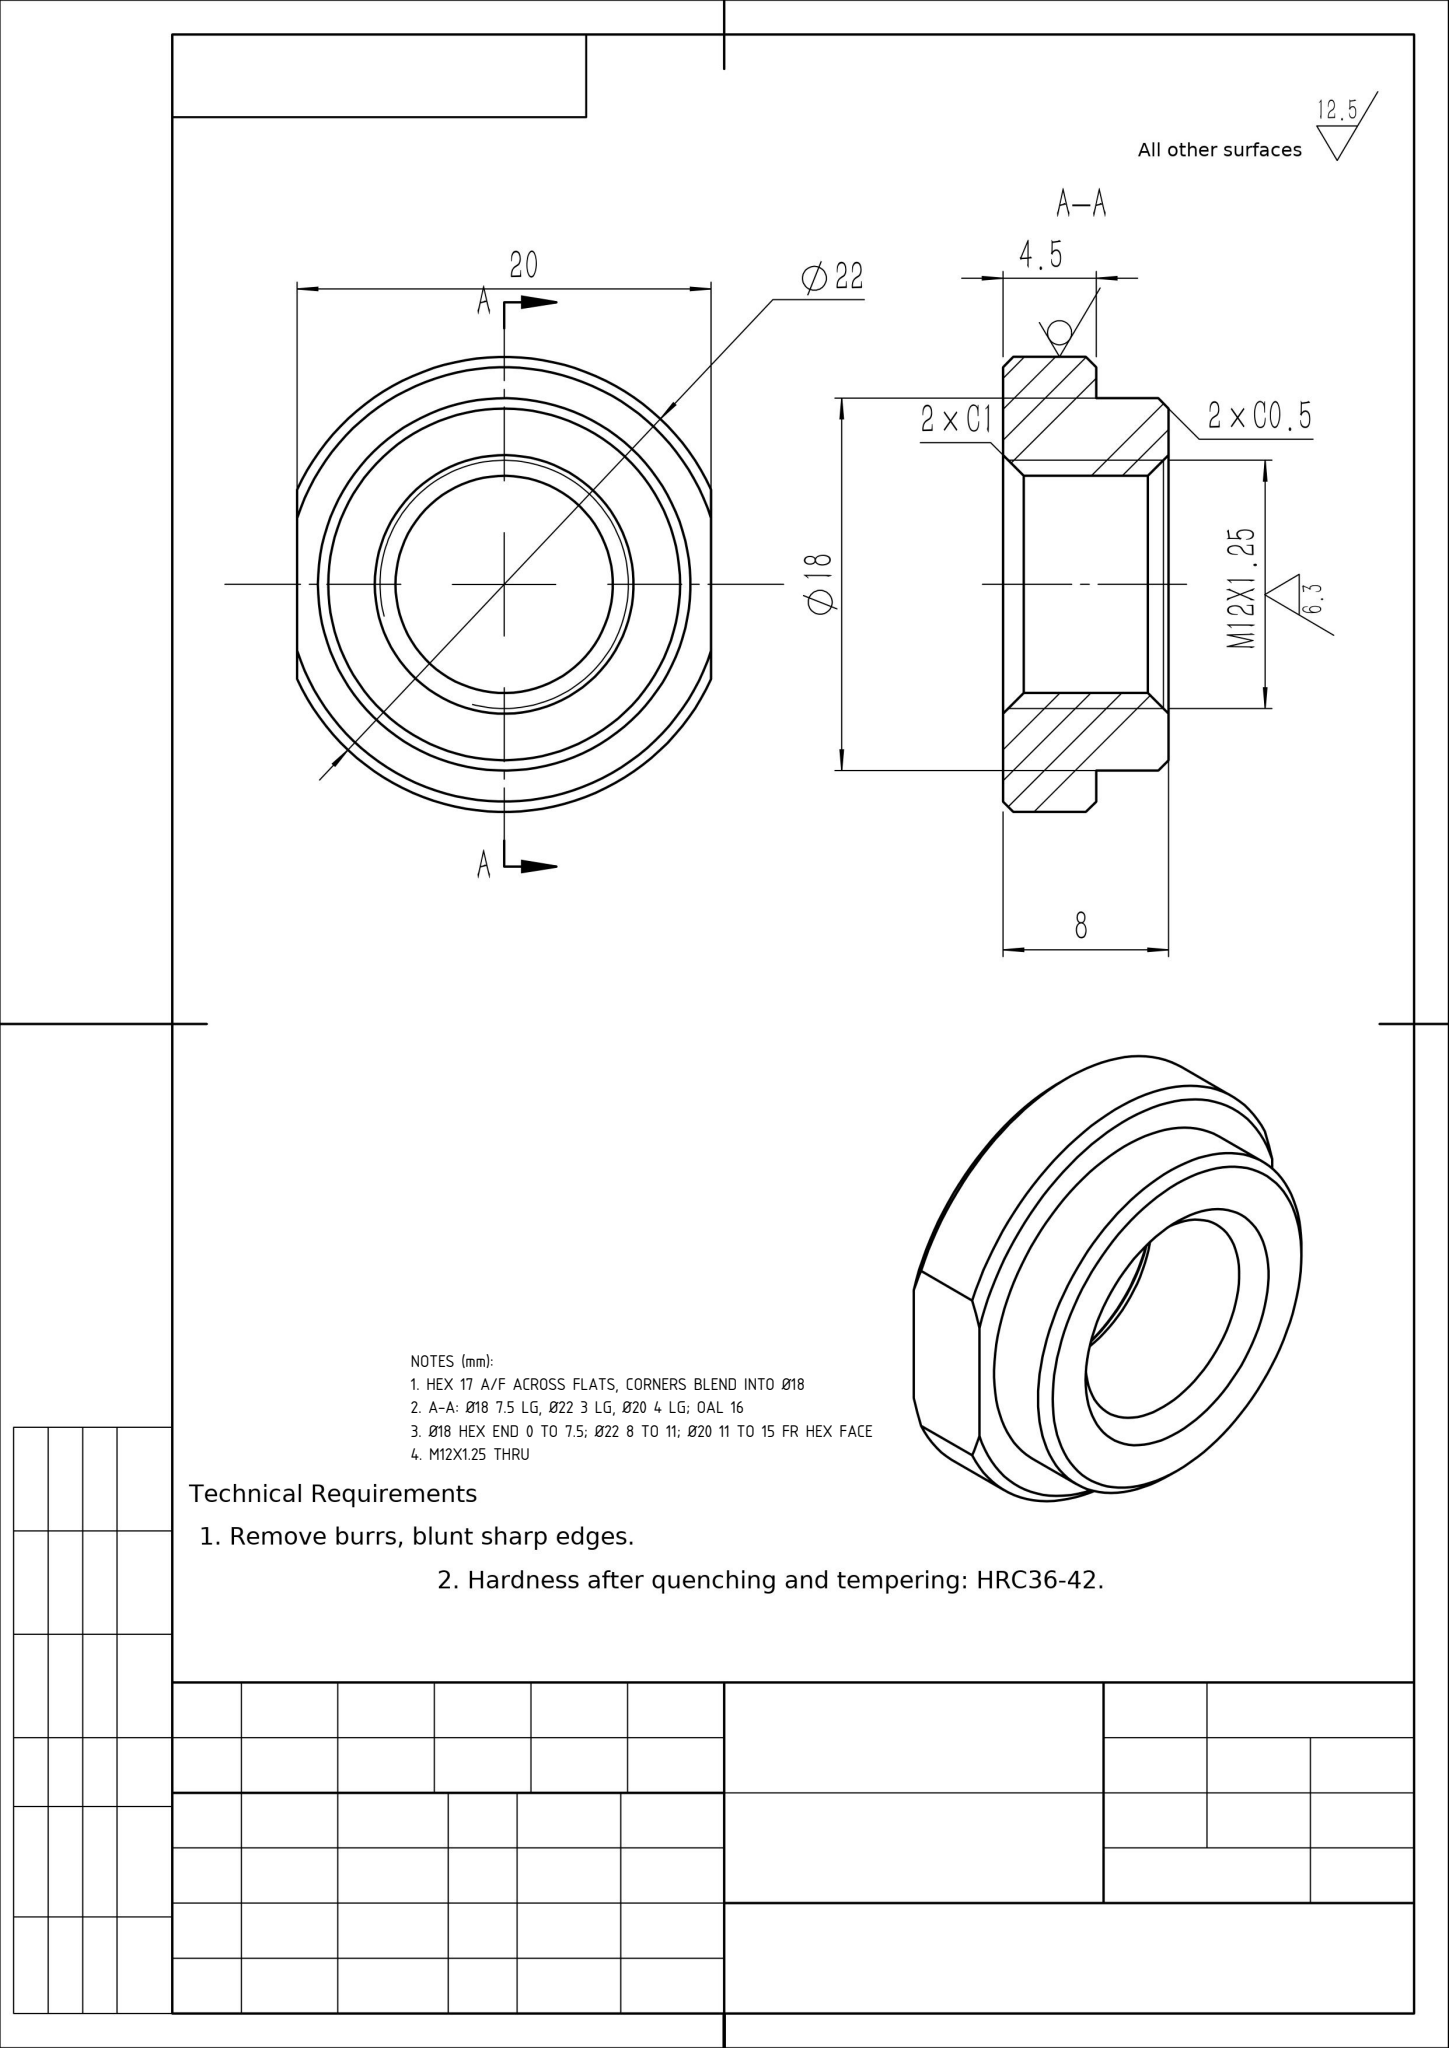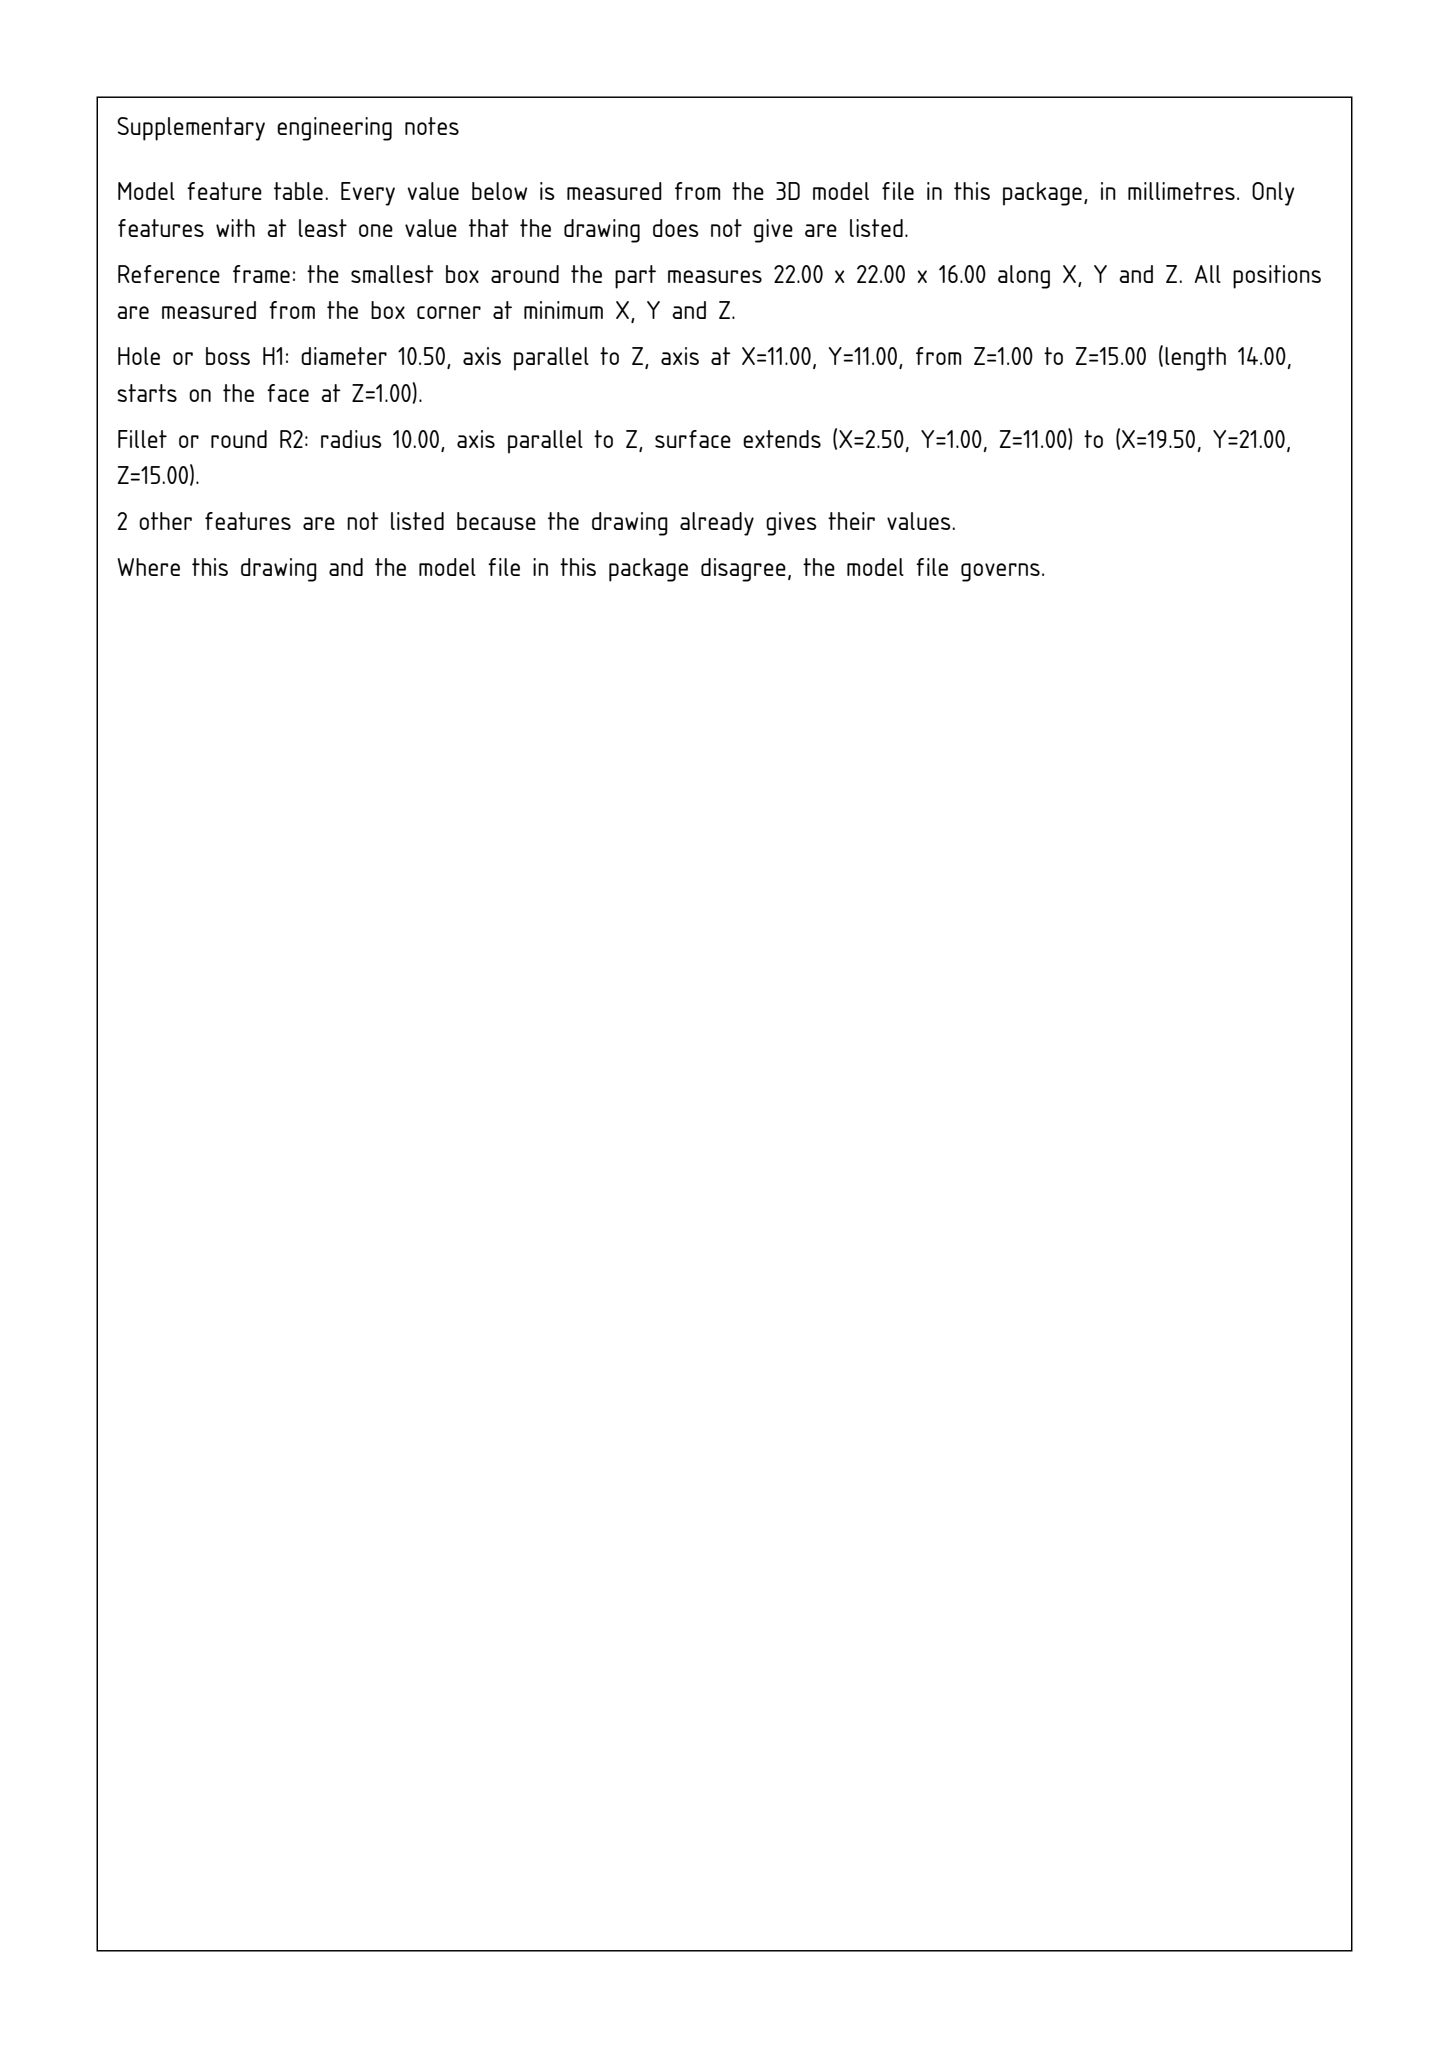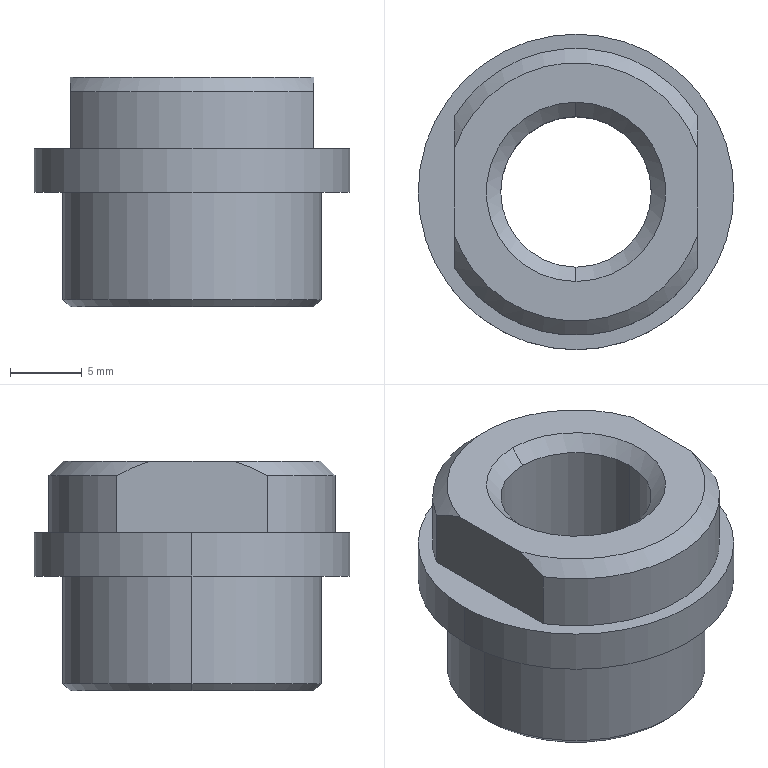Part | SolidWorks | mm | 1 solid | 22 faces | box 22 x 22 x 16 mm | volume 3192 mm3 | cone 8 | cylinder 8 | plane 6 | commonest cylinder face diameters 10.5 x2 18 x2 22 x2 20 x2
Drawing notes:
HEX 17 A/F ACROSS FLATS, CORNERS BLEND INTO Ø18 | from the solid: axis_planes x=2.5 and x=19.5 -> 17 across flats on Ø18 (dia 18) section
A-A: Ø18 7.5 LG, Ø22 3 LG, Ø20 4 LG; OAL 16 | from the solid: cylinders dia18 L7.5, dia22 L3, dia20 L4; bbox z=16.001
Ø18 HEX END 0 TO 7.5; Ø22 8 TO 11; Ø20 11 TO 15 FR HEX FACE | from the solid: z planes 0, 8, 11, 16 with cyl lengths 7.5 / 3 / 4 from z=0 end face
M12X1.25 THRU | from the solid: Ø10.5 bore L14 + C1 both ends = 16 = full part length
build123d program:
from build123d import *

# Parameters (mm, degrees)
CHAMFER1_SIZE               = 1
CHAMFER2_SIZE               = 0.5
CUT_EXTRUDE1_REACH          = 24.316
SKETCH2_W                   = 1.5
SKETCH2_H                   = 20
M12X1_25_TAPPED_HOLE1_D     = 10.5
M12X1_25_TAPPED_HOLE1_DEPTH = 27.75
M12X1_25_TAPPED_HOLE1_TIP   = 3.155
CHAMFER3_SIZE               = 1


with BuildPart() as part:
    # Sketch1 → Revolve1 (revolve)
    with BuildSketch(Plane(origin=(0, 0, 0), x_dir=(0, 0, -1), z_dir=(1, 0, 0)), mode=Mode.PRIVATE) as revolve1_sk:
        Polygon((0, 0), (0, 10), (5, 10), (5, 11), (8, 11), (8, 9), (16, 9), (16, 0), align=None)
    revolve(revolve1_sk.sketch.rotate(Axis((0, 0, -16), (0, 0, 1)), 90), axis=Axis((0, 0, -16), (0, 0, 1)))

    # Chamfer1
    chamfer1_edges = [part.edges().sort_by_distance(p)[0] for p in [
        (10, 0, 0),
    ]]
    chamfer(chamfer1_edges, length=CHAMFER1_SIZE)

    # Chamfer2
    chamfer2_edges = [part.edges().sort_by_distance(p)[0] for p in [
        (9, 0, -16),
    ]]
    chamfer(chamfer2_edges, length=CHAMFER2_SIZE)

    # Cut-Extrude1: up to this face of the body (flat: up to its plane)
    cut_extrude1_end = Plane(part.part.faces().sort_by_distance((10.311, 0, -5))[0])
    # Sketch2 → Cut-Extrude1 (cut, up to the picked face)
    with BuildSketch(Plane.XY, mode=Mode.PRIVATE) as cut_extrude1_sk1:
        with Locations((-9.25, 0)):
            Rectangle(SKETCH2_W, SKETCH2_H)
    cut_extrude1_tool1 = split(extrude(cut_extrude1_sk1.sketch, amount=-CUT_EXTRUDE1_REACH, mode=Mode.PRIVATE), bisect_by=cut_extrude1_end, keep=Keep.BOTH, mode=Mode.PRIVATE)
    cut_extrude1 = cut_extrude1_tool1.solids().sort_by(Axis((-9.25, 0, 0), (0, 0, -1)))[0]
    add(cut_extrude1, mode=Mode.SUBTRACT)

    # Mirror1: Cut-Extrude1 across plane
    add(cut_extrude1.mirror(Plane(origin=(0, 0, 0), x_dir=(0, 0, 1), z_dir=(1, 0, 0))), mode=Mode.SUBTRACT)

    # M12x1.25 Tapped Hole1
    with Locations(Plane.XY):
        with Locations((0, 0)):
            Hole(M12X1_25_TAPPED_HOLE1_D / 2, depth=M12X1_25_TAPPED_HOLE1_DEPTH)
            with Locations((0, 0, -(M12X1_25_TAPPED_HOLE1_DEPTH + M12X1_25_TAPPED_HOLE1_TIP / 2))):  # 118° drill point
                Cone(0, M12X1_25_TAPPED_HOLE1_D / 2, M12X1_25_TAPPED_HOLE1_TIP, mode=Mode.SUBTRACT)

    # Chamfer3
    chamfer3_edges = [part.edges().sort_by_distance(p)[0] for p in [
        (5.25, 0, -16),
        (5.25, 0, 0),
    ]]
    chamfer(chamfer3_edges, length=CHAMFER3_SIZE)


solid = part.part
STEP:
#1=CARTESIAN_POINT('',(0.,-5.25,-15.));
#2=VERTEX_POINT('',#1);
#3=CARTESIAN_POINT('',(-5.25,0.,-15.));
#4=VERTEX_POINT('',#3);
#5=CARTESIAN_POINT('',(0.,0.,-15.));
#6=DIRECTION('',(0.,0.,-1.));
#7=DIRECTION('',(0.,1.,0.));
#8=AXIS2_PLACEMENT_3D('',#5,#6,#7);
#9=CIRCLE('',#8,5.25);
#10=EDGE_CURVE('',#2,#4,#9,.T.);
#11=ORIENTED_EDGE('',*,*,#10,.F.);
#12=CARTESIAN_POINT('',(0.,-6.25,-16.));
#13=VERTEX_POINT('',#12);
#14=CARTESIAN_POINT('',(0.,-5.25,-15.));
#15=DIRECTION('',(0.,-0.7071,-0.7071));
#16=VECTOR('',#15,1000.);
#17=LINE('',#14,#16);
#18=EDGE_CURVE('',#2,#13,#17,.T.);
#19=ORIENTED_EDGE('',*,*,#18,.T.);
#20=CARTESIAN_POINT('',(0.,6.25,-16.));
#21=VERTEX_POINT('',#20);
#22=CARTESIAN_POINT('',(0.,0.,-16.));
#23=DIRECTION('',(-0.,-0.,1.));
#24=DIRECTION('',(0.,1.,0.));
#25=AXIS2_PLACEMENT_3D('',#22,#23,#24);
#26=CIRCLE('',#25,6.25);
#27=EDGE_CURVE('',#21,#13,#26,.T.);
#28=ORIENTED_EDGE('',*,*,#27,.F.);
#29=CARTESIAN_POINT('',(0.,5.25,-15.));
#30=VERTEX_POINT('',#29);
#31=CARTESIAN_POINT('',(0.,5.25,-15.));
#32=DIRECTION('',(0.,0.7071,-0.7071));
#33=VECTOR('',#32,1000.);
#34=LINE('',#31,#33);
#35=EDGE_CURVE('',#30,#21,#34,.T.);
#36=ORIENTED_EDGE('',*,*,#35,.F.);
#37=CARTESIAN_POINT('',(0.,0.,-15.));
#38=DIRECTION('',(0.,0.,-1.));
#39=DIRECTION('',(0.,1.,0.));
#40=AXIS2_PLACEMENT_3D('',#37,#38,#39);
#41=CIRCLE('',#40,5.25);
#42=EDGE_CURVE('',#4,#30,#41,.T.);
#43=ORIENTED_EDGE('',*,*,#42,.F.);
#44=EDGE_LOOP('',(#11,#19,#28,#36,#43));
#45=FACE_OUTER_BOUND('',#44,.T.);
#46=CARTESIAN_POINT('',(0.,0.,-15.));
#47=DIRECTION('',(0.,0.,-1.));
#48=DIRECTION('',(0.,1.,0.));
#49=AXIS2_PLACEMENT_3D('',#46,#47,#48);
#50=CONICAL_SURFACE('',#49,5.25,0.7854);
#51=ADVANCED_FACE('',(#45),#50,.F.);
#52=CARTESIAN_POINT('',(0.,5.25,-1.));
#53=VERTEX_POINT('',#52);
#54=CARTESIAN_POINT('',(-5.25,0.,-1.));
#55=VERTEX_POINT('',#54);
#56=CARTESIAN_POINT('',(0.,0.,-1.));
#57=DIRECTION('',(-0.,-0.,1.));
#58=DIRECTION('',(0.,-1.,0.));
#59=AXIS2_PLACEMENT_3D('',#56,#57,#58);
#60=CIRCLE('',#59,5.25);
#61=EDGE_CURVE('',#53,#55,#60,.T.);
#62=ORIENTED_EDGE('',*,*,#61,.F.);
#63=CARTESIAN_POINT('',(0.,6.25,0.));
#64=VERTEX_POINT('',#63);
#65=CARTESIAN_POINT('',(0.,5.25,-1.));
#66=DIRECTION('',(0.,0.7071,0.7071));
#67=VECTOR('',#66,1000.);
#68=LINE('',#65,#67);
#69=EDGE_CURVE('',#53,#64,#68,.T.);
#70=ORIENTED_EDGE('',*,*,#69,.T.);
#71=CARTESIAN_POINT('',(0.,-6.25,0.));
#72=VERTEX_POINT('',#71);
#73=CARTESIAN_POINT('',(0.,0.,0.));
#74=DIRECTION('',(0.,0.,-1.));
#75=DIRECTION('',(0.,-1.,-0.));
#76=AXIS2_PLACEMENT_3D('',#73,#74,#75);
#77=CIRCLE('',#76,6.25);
#78=EDGE_CURVE('',#72,#64,#77,.T.);
#79=ORIENTED_EDGE('',*,*,#78,.F.);
#80=CARTESIAN_POINT('',(0.,-5.25,-1.));
#81=VERTEX_POINT('',#80);
#82=CARTESIAN_POINT('',(0.,-5.25,-1.));
#83=DIRECTION('',(-0.,-0.7071,0.7071));
#84=VECTOR('',#83,1000.);
#85=LINE('',#82,#84);
#86=EDGE_CURVE('',#81,#72,#85,.T.);
#87=ORIENTED_EDGE('',*,*,#86,.F.);
#88=CARTESIAN_POINT('',(0.,0.,-1.));
#89=DIRECTION('',(-0.,-0.,1.));
#90=DIRECTION('',(0.,-1.,0.));
#91=AXIS2_PLACEMENT_3D('',#88,#89,#90);
#92=CIRCLE('',#91,5.25);
#93=EDGE_CURVE('',#55,#81,#92,.T.);
#94=ORIENTED_EDGE('',*,*,#93,.F.);
#95=EDGE_LOOP('',(#62,#70,#79,#87,#94));
#96=FACE_OUTER_BOUND('',#95,.T.);
#97=CARTESIAN_POINT('',(0.,0.,-1.));
#98=DIRECTION('',(-0.,-0.,1.));
#99=DIRECTION('',(0.,-1.,0.));
#100=AXIS2_PLACEMENT_3D('',#97,#98,#99);
#101=CONICAL_SURFACE('',#100,5.25,0.7854);
#102=ADVANCED_FACE('',(#96),#101,.F.);
#103=CARTESIAN_POINT('',(5.25,-0.,-15.));
#104=VERTEX_POINT('',#103);
#105=CARTESIAN_POINT('',(0.,0.,-15.));
#106=DIRECTION('',(0.,0.,-1.));
#107=DIRECTION('',(0.,1.,0.));
#108=AXIS2_PLACEMENT_3D('',#105,#106,#107);
#109=CIRCLE('',#108,5.25);
#110=EDGE_CURVE('',#104,#2,#109,.T.);
#111=ORIENTED_EDGE('',*,*,#110,.T.);
#112=ORIENTED_EDGE('',*,*,#10,.T.);
#113=CARTESIAN_POINT('',(-5.25,0.,0.));
#114=DIRECTION('',(-0.,-0.,1.));
#115=VECTOR('',#114,1000.);
#116=LINE('',#113,#115);
#117=EDGE_CURVE('',#4,#55,#116,.T.);
#118=ORIENTED_EDGE('',*,*,#117,.T.);
#119=ORIENTED_EDGE('',*,*,#93,.T.);
#120=CARTESIAN_POINT('',(5.25,-0.,-1.));
#121=VERTEX_POINT('',#120);
#122=CARTESIAN_POINT('',(0.,0.,-1.));
#123=DIRECTION('',(-0.,-0.,1.));
#124=DIRECTION('',(0.,-1.,0.));
#125=AXIS2_PLACEMENT_3D('',#122,#123,#124);
#126=CIRCLE('',#125,5.25);
#127=EDGE_CURVE('',#81,#121,#126,.T.);
#128=ORIENTED_EDGE('',*,*,#127,.T.);
#129=CARTESIAN_POINT('',(5.25,-0.,-0.));
#130=DIRECTION('',(-0.,-0.,1.));
#131=VECTOR('',#130,1000.);
#132=LINE('',#129,#131);
#133=EDGE_CURVE('',#104,#121,#132,.T.);
#134=ORIENTED_EDGE('',*,*,#133,.F.);
#135=EDGE_LOOP('',(#111,#112,#118,#119,#128,#134));
#136=FACE_OUTER_BOUND('',#135,.T.);
#137=CARTESIAN_POINT('',(0.,0.,0.));
#138=DIRECTION('',(-0.,-0.,1.));
#139=DIRECTION('',(1.,-0.,-0.));
#140=AXIS2_PLACEMENT_3D('',#137,#138,#139);
#141=CYLINDRICAL_SURFACE('',#140,5.25);
#142=ADVANCED_FACE('',(#136),#141,.F.);
#143=CARTESIAN_POINT('',(-8.5,0.,-16.));
#144=VERTEX_POINT('',#143);
#145=CARTESIAN_POINT('',(8.5,-0.,-16.));
#146=VERTEX_POINT('',#145);
#147=CARTESIAN_POINT('',(0.,0.,-16.));
#148=DIRECTION('',(0.,0.,-1.));
#149=DIRECTION('',(-1.,0.,0.));
#150=AXIS2_PLACEMENT_3D('',#147,#148,#149);
#151=CIRCLE('',#150,8.5);
#152=EDGE_CURVE('',#144,#146,#151,.T.);
#153=ORIENTED_EDGE('',*,*,#152,.F.);
#154=CARTESIAN_POINT('',(-9.,0.,-15.5));
#155=VERTEX_POINT('',#154);
#156=CARTESIAN_POINT('',(-8.5,0.,-16.));
#157=DIRECTION('',(-0.7071,0.,0.7071));
#158=VECTOR('',#157,1000.);
#159=LINE('',#156,#158);
#160=EDGE_CURVE('',#144,#155,#159,.T.);
#161=ORIENTED_EDGE('',*,*,#160,.T.);
#162=CARTESIAN_POINT('',(9.,-0.,-15.5));
#163=VERTEX_POINT('',#162);
#164=CARTESIAN_POINT('',(0.,0.,-15.5));
#165=DIRECTION('',(-0.,-0.,1.));
#166=DIRECTION('',(-1.,0.,0.));
#167=AXIS2_PLACEMENT_3D('',#164,#165,#166);
#168=CIRCLE('',#167,9.);
#169=EDGE_CURVE('',#163,#155,#168,.T.);
#170=ORIENTED_EDGE('',*,*,#169,.F.);
#171=CARTESIAN_POINT('',(8.5,-0.,-16.));
#172=DIRECTION('',(0.7071,-0.,0.7071));
#173=VECTOR('',#172,1000.);
#174=LINE('',#171,#173);
#175=EDGE_CURVE('',#146,#163,#174,.T.);
#176=ORIENTED_EDGE('',*,*,#175,.F.);
#177=EDGE_LOOP('',(#153,#161,#170,#176));
#178=FACE_OUTER_BOUND('',#177,.T.);
#179=CARTESIAN_POINT('',(0.,0.,-16.));
#180=DIRECTION('',(-0.,-0.,1.));
#181=DIRECTION('',(1.,-0.,0.));
#182=AXIS2_PLACEMENT_3D('',#179,#180,#181);
#183=CONICAL_SURFACE('',#182,8.5,0.7854);
#184=ADVANCED_FACE('',(#178),#183,.T.);
#185=CARTESIAN_POINT('',(-9.,0.,-8.));
#186=VERTEX_POINT('',#185);
#187=CARTESIAN_POINT('',(9.,-0.,-8.));
#188=VERTEX_POINT('',#187);
#189=CARTESIAN_POINT('',(0.,0.,-8.));
#190=DIRECTION('',(0.,0.,-1.));
#191=DIRECTION('',(-1.,0.,0.));
#192=AXIS2_PLACEMENT_3D('',#189,#190,#191);
#193=CIRCLE('',#192,9.);
#194=EDGE_CURVE('',#186,#188,#193,.T.);
#195=ORIENTED_EDGE('',*,*,#194,.T.);
#196=CARTESIAN_POINT('',(9.,-0.,-16.));
#197=DIRECTION('',(0.,0.,-1.));
#198=VECTOR('',#197,1000.);
#199=LINE('',#196,#198);
#200=EDGE_CURVE('',#188,#163,#199,.T.);
#201=ORIENTED_EDGE('',*,*,#200,.T.);
#202=ORIENTED_EDGE('',*,*,#169,.T.);
#203=CARTESIAN_POINT('',(-9.,0.,-16.));
#204=DIRECTION('',(0.,0.,-1.));
#205=VECTOR('',#204,1000.);
#206=LINE('',#203,#205);
#207=EDGE_CURVE('',#186,#155,#206,.T.);
#208=ORIENTED_EDGE('',*,*,#207,.F.);
#209=EDGE_LOOP('',(#195,#201,#202,#208));
#210=FACE_OUTER_BOUND('',#209,.T.);
#211=CARTESIAN_POINT('',(0.,0.,-16.));
#212=DIRECTION('',(0.,0.,-1.));
#213=DIRECTION('',(-1.,0.,0.));
#214=AXIS2_PLACEMENT_3D('',#211,#212,#213);
#215=CYLINDRICAL_SURFACE('',#214,9.);
#216=ADVANCED_FACE('',(#210),#215,.T.);
#217=CARTESIAN_POINT('',(-11.,0.,-5.));
#218=VERTEX_POINT('',#217);
#219=CARTESIAN_POINT('',(11.,-0.,-5.));
#220=VERTEX_POINT('',#219);
#221=CARTESIAN_POINT('',(0.,0.,-5.));
#222=DIRECTION('',(0.,0.,-1.));
#223=DIRECTION('',(-1.,0.,0.));
#224=AXIS2_PLACEMENT_3D('',#221,#222,#223);
#225=CIRCLE('',#224,11.);
#226=EDGE_CURVE('',#218,#220,#225,.T.);
#227=ORIENTED_EDGE('',*,*,#226,.T.);
#228=CARTESIAN_POINT('',(11.,-0.,-8.));
#229=VERTEX_POINT('',#228);
#230=CARTESIAN_POINT('',(11.,-0.,-16.));
#231=DIRECTION('',(0.,0.,-1.));
#232=VECTOR('',#231,1000.);
#233=LINE('',#230,#232);
#234=EDGE_CURVE('',#220,#229,#233,.T.);
#235=ORIENTED_EDGE('',*,*,#234,.T.);
#236=CARTESIAN_POINT('',(-11.,0.,-8.));
#237=VERTEX_POINT('',#236);
#238=CARTESIAN_POINT('',(0.,0.,-8.));
#239=DIRECTION('',(0.,0.,-1.));
#240=DIRECTION('',(-1.,0.,0.));
#241=AXIS2_PLACEMENT_3D('',#238,#239,#240);
#242=CIRCLE('',#241,11.);
#243=EDGE_CURVE('',#237,#229,#242,.T.);
#244=ORIENTED_EDGE('',*,*,#243,.F.);
#245=CARTESIAN_POINT('',(-11.,0.,-16.));
#246=DIRECTION('',(0.,0.,-1.));
#247=VECTOR('',#246,1000.);
#248=LINE('',#245,#247);
#249=EDGE_CURVE('',#218,#237,#248,.T.);
#250=ORIENTED_EDGE('',*,*,#249,.F.);
#251=EDGE_LOOP('',(#227,#235,#244,#250));
#252=FACE_OUTER_BOUND('',#251,.T.);
#253=CARTESIAN_POINT('',(0.,0.,-16.));
#254=DIRECTION('',(0.,0.,-1.));
#255=DIRECTION('',(-1.,0.,0.));
#256=AXIS2_PLACEMENT_3D('',#253,#254,#255);
#257=CYLINDRICAL_SURFACE('',#256,11.);
#258=ADVANCED_FACE('',(#252),#257,.T.);
#259=ORIENTED_EDGE('',*,*,#78,.T.);
#260=CARTESIAN_POINT('',(0.,0.,0.));
#261=DIRECTION('',(0.,0.,-1.));
#262=DIRECTION('',(0.,-1.,-0.));
#263=AXIS2_PLACEMENT_3D('',#260,#261,#262);
#264=CIRCLE('',#263,6.25);
#265=EDGE_CURVE('',#64,#72,#264,.T.);
#266=ORIENTED_EDGE('',*,*,#265,.T.);
#267=EDGE_LOOP('',(#259,#266));
#268=FACE_BOUND('',#267,.T.);
#269=CARTESIAN_POINT('',(-8.5,-2.958,0.));
#270=VERTEX_POINT('',#269);
#271=CARTESIAN_POINT('',(8.5,-2.958,0.));
#272=VERTEX_POINT('',#271);
#273=CARTESIAN_POINT('',(0.,0.,0.));
#274=DIRECTION('',(-0.,-0.,1.));
#275=DIRECTION('',(1.,-0.,-0.));
#276=AXIS2_PLACEMENT_3D('',#273,#274,#275);
#277=CIRCLE('',#276,9.);
#278=EDGE_CURVE('',#270,#272,#277,.T.);
#279=ORIENTED_EDGE('',*,*,#278,.T.);
#280=CARTESIAN_POINT('',(8.5,2.958,0.));
#281=VERTEX_POINT('',#280);
#282=CARTESIAN_POINT('',(8.5,10.,0.));
#283=DIRECTION('',(-0.,1.,-0.));
#284=VECTOR('',#283,1000.);
#285=LINE('',#282,#284);
#286=EDGE_CURVE('',#272,#281,#285,.T.);
#287=ORIENTED_EDGE('',*,*,#286,.T.);
#288=CARTESIAN_POINT('',(-8.5,2.958,0.));
#289=VERTEX_POINT('',#288);
#290=CARTESIAN_POINT('',(0.,0.,0.));
#291=DIRECTION('',(-0.,-0.,1.));
#292=DIRECTION('',(1.,-0.,-0.));
#293=AXIS2_PLACEMENT_3D('',#290,#291,#292);
#294=CIRCLE('',#293,9.);
#295=EDGE_CURVE('',#281,#289,#294,.T.);
#296=ORIENTED_EDGE('',*,*,#295,.T.);
#297=CARTESIAN_POINT('',(-8.5,10.,0.));
#298=DIRECTION('',(-0.,1.,-0.));
#299=VECTOR('',#298,1000.);
#300=LINE('',#297,#299);
#301=EDGE_CURVE('',#270,#289,#300,.T.);
#302=ORIENTED_EDGE('',*,*,#301,.F.);
#303=EDGE_LOOP('',(#279,#287,#296,#302));
#304=FACE_OUTER_BOUND('',#303,.T.);
#305=CARTESIAN_POINT('',(0.,0.,0.));
#306=DIRECTION('',(0.,-0.,1.));
#307=DIRECTION('',(1.,-0.,-0.));
#308=AXIS2_PLACEMENT_3D('',#305,#306,#307);
#309=PLANE('',#308);
#310=ADVANCED_FACE('',(#268,#304),#309,.T.);
#311=CARTESIAN_POINT('',(8.5,-5.268,-5.));
#312=VERTEX_POINT('',#311);
#313=CARTESIAN_POINT('',(-8.5,-5.268,-5.));
#314=VERTEX_POINT('',#313);
#315=CARTESIAN_POINT('',(0.,0.,-5.));
#316=DIRECTION('',(0.,0.,-1.));
#317=DIRECTION('',(-1.,0.,0.));
#318=AXIS2_PLACEMENT_3D('',#315,#316,#317);
#319=CIRCLE('',#318,10.);
#320=EDGE_CURVE('',#312,#314,#319,.T.);
#321=ORIENTED_EDGE('',*,*,#320,.F.);
#322=CARTESIAN_POINT('',(8.5,-5.268,-1.));
#323=VERTEX_POINT('',#322);
#324=CARTESIAN_POINT('',(8.5,-5.268,-16.));
#325=DIRECTION('',(-0.,-0.,1.));
#326=VECTOR('',#325,1000.);
#327=LINE('',#324,#326);
#328=EDGE_CURVE('',#312,#323,#327,.T.);
#329=ORIENTED_EDGE('',*,*,#328,.T.);
#330=CARTESIAN_POINT('',(-8.5,-5.268,-1.));
#331=VERTEX_POINT('',#330);
#332=CARTESIAN_POINT('',(0.,0.,-1.));
#333=DIRECTION('',(0.,0.,-1.));
#334=DIRECTION('',(1.,-0.,0.));
#335=AXIS2_PLACEMENT_3D('',#332,#333,#334);
#336=CIRCLE('',#335,10.);
#337=EDGE_CURVE('',#323,#331,#336,.T.);
#338=ORIENTED_EDGE('',*,*,#337,.T.);
#339=CARTESIAN_POINT('',(-8.5,-5.268,-16.));
#340=DIRECTION('',(-0.,-0.,1.));
#341=VECTOR('',#340,1000.);
#342=LINE('',#339,#341);
#343=EDGE_CURVE('',#314,#331,#342,.T.);
#344=ORIENTED_EDGE('',*,*,#343,.F.);
#345=EDGE_LOOP('',(#321,#329,#338,#344));
#346=FACE_OUTER_BOUND('',#345,.T.);
#347=CARTESIAN_POINT('',(0.,0.,-16.));
#348=DIRECTION('',(0.,0.,-1.));
#349=DIRECTION('',(-1.,0.,0.));
#350=AXIS2_PLACEMENT_3D('',#347,#348,#349);
#351=CYLINDRICAL_SURFACE('',#350,10.);
#352=ADVANCED_FACE('',(#346),#351,.T.);
#353=CARTESIAN_POINT('',(-8.5,5.268,-1.));
#354=VERTEX_POINT('',#353);
#355=CARTESIAN_POINT('',(8.5,5.268,-1.));
#356=VERTEX_POINT('',#355);
#357=CARTESIAN_POINT('',(0.,0.,-1.));
#358=DIRECTION('',(0.,0.,-1.));
#359=DIRECTION('',(1.,-0.,0.));
#360=AXIS2_PLACEMENT_3D('',#357,#358,#359);
#361=CIRCLE('',#360,10.);
#362=EDGE_CURVE('',#354,#356,#361,.T.);
#363=ORIENTED_EDGE('',*,*,#362,.T.);
#364=CARTESIAN_POINT('',(8.5,5.268,-5.));
#365=VERTEX_POINT('',#364);
#366=CARTESIAN_POINT('',(8.5,5.268,-16.));
#367=DIRECTION('',(0.,0.,-1.));
#368=VECTOR('',#367,1000.);
#369=LINE('',#366,#368);
#370=EDGE_CURVE('',#356,#365,#369,.T.);
#371=ORIENTED_EDGE('',*,*,#370,.T.);
#372=CARTESIAN_POINT('',(-8.5,5.268,-5.));
#373=VERTEX_POINT('',#372);
#374=CARTESIAN_POINT('',(0.,0.,-5.));
#375=DIRECTION('',(0.,0.,-1.));
#376=DIRECTION('',(-1.,0.,0.));
#377=AXIS2_PLACEMENT_3D('',#374,#375,#376);
#378=CIRCLE('',#377,10.);
#379=EDGE_CURVE('',#373,#365,#378,.T.);
#380=ORIENTED_EDGE('',*,*,#379,.F.);
#381=CARTESIAN_POINT('',(-8.5,5.268,-16.));
#382=DIRECTION('',(0.,0.,-1.));
#383=VECTOR('',#382,1000.);
#384=LINE('',#381,#383);
#385=EDGE_CURVE('',#354,#373,#384,.T.);
#386=ORIENTED_EDGE('',*,*,#385,.F.);
#387=EDGE_LOOP('',(#363,#371,#380,#386));
#388=FACE_OUTER_BOUND('',#387,.T.);
#389=CARTESIAN_POINT('',(0.,0.,-16.));
#390=DIRECTION('',(0.,0.,-1.));
#391=DIRECTION('',(-1.,0.,0.));
#392=AXIS2_PLACEMENT_3D('',#389,#390,#391);
#393=CYLINDRICAL_SURFACE('',#392,10.);
#394=ADVANCED_FACE('',(#388),#393,.T.);
#395=ORIENTED_EDGE('',*,*,#337,.F.);
#396=CARTESIAN_POINT('',(8.5,-5.268,-1.));
#397=CARTESIAN_POINT('',(8.5,-4.525,-0.6089));
#398=CARTESIAN_POINT('',(8.5,-3.761,-0.2639));
#399=CARTESIAN_POINT('',(8.5,-2.958,0.));
#400=B_SPLINE_CURVE_WITH_KNOTS('',3,(#396,#397,#398,#399),.UNSPECIFIED.,.F.,.F.,(4,4),(0.01929,0.02181),.UNSPECIFIED.);
#401=EDGE_CURVE('',#323,#272,#400,.T.);
#402=ORIENTED_EDGE('',*,*,#401,.T.);
#403=ORIENTED_EDGE('',*,*,#278,.F.);
#404=CARTESIAN_POINT('',(-8.5,-5.268,-1.));
#405=CARTESIAN_POINT('',(-8.5,-4.525,-0.6089));
#406=CARTESIAN_POINT('',(-8.5,-3.761,-0.2639));
#407=CARTESIAN_POINT('',(-8.5,-2.958,0.));
#408=B_SPLINE_CURVE_WITH_KNOTS('',3,(#404,#405,#406,#407),.UNSPECIFIED.,.F.,.F.,(4,4),(0.01929,0.02181),.UNSPECIFIED.);
#409=EDGE_CURVE('',#331,#270,#408,.T.);
#410=ORIENTED_EDGE('',*,*,#409,.F.);
#411=EDGE_LOOP('',(#395,#402,#403,#410));
#412=FACE_OUTER_BOUND('',#411,.T.);
#413=CARTESIAN_POINT('',(0.,0.,-1.));
#414=DIRECTION('',(0.,0.,-1.));
#415=DIRECTION('',(-1.,0.,0.));
#416=AXIS2_PLACEMENT_3D('',#413,#414,#415);
#417=CONICAL_SURFACE('',#416,10.,0.7854);
#418=ADVANCED_FACE('',(#412),#417,.T.);
#419=ORIENTED_EDGE('',*,*,#295,.F.);
#420=CARTESIAN_POINT('',(8.5,2.958,0.));
#421=CARTESIAN_POINT('',(8.5,3.36,-0.132));
#422=CARTESIAN_POINT('',(8.5,3.755,-0.2859));
#423=CARTESIAN_POINT('',(8.5,4.523,-0.6224));
#424=CARTESIAN_POINT('',(8.5,4.899,-0.8056));
#425=CARTESIAN_POINT('',(8.5,5.268,-1.));
#426=B_SPLINE_CURVE_WITH_KNOTS('',3,(#420,#421,#422,#423,#424,#425),.UNSPECIFIED.,.F.,.F.,(4,2,4),(0.02784,0.02911,0.03037),.UNSPECIFIED.);
#427=EDGE_CURVE('',#281,#356,#426,.T.);
#428=ORIENTED_EDGE('',*,*,#427,.T.);
#429=ORIENTED_EDGE('',*,*,#362,.F.);
#430=CARTESIAN_POINT('',(-8.5,2.958,0.));
#431=CARTESIAN_POINT('',(-8.5,3.36,-0.132));
#432=CARTESIAN_POINT('',(-8.5,3.755,-0.2859));
#433=CARTESIAN_POINT('',(-8.5,4.523,-0.6224));
#434=CARTESIAN_POINT('',(-8.5,4.899,-0.8056));
#435=CARTESIAN_POINT('',(-8.5,5.268,-1.));
#436=B_SPLINE_CURVE_WITH_KNOTS('',3,(#430,#431,#432,#433,#434,#435),.UNSPECIFIED.,.F.,.F.,(4,2,4),(0.02784,0.02911,0.03037),.UNSPECIFIED.);
#437=EDGE_CURVE('',#289,#354,#436,.T.);
#438=ORIENTED_EDGE('',*,*,#437,.F.);
#439=EDGE_LOOP('',(#419,#428,#429,#438));
#440=FACE_OUTER_BOUND('',#439,.T.);
#441=CARTESIAN_POINT('',(0.,0.,-1.));
#442=DIRECTION('',(0.,0.,-1.));
#443=DIRECTION('',(-1.,0.,0.));
#444=AXIS2_PLACEMENT_3D('',#441,#442,#443);
#445=CONICAL_SURFACE('',#444,10.,0.7854);
#446=ADVANCED_FACE('',(#440),#445,.T.);
#447=CARTESIAN_POINT('',(8.5,10.,-5.));
#448=DIRECTION('',(0.,-1.,0.));
#449=VECTOR('',#448,1000.);
#450=LINE('',#447,#449);
#451=EDGE_CURVE('',#365,#312,#450,.T.);
#452=ORIENTED_EDGE('',*,*,#451,.T.);
#453=ORIENTED_EDGE('',*,*,#320,.T.);
#454=CARTESIAN_POINT('',(-8.5,10.,-5.));
#455=DIRECTION('',(0.,-1.,0.));
#456=VECTOR('',#455,1000.);
#457=LINE('',#454,#456);
#458=EDGE_CURVE('',#373,#314,#457,.T.);
#459=ORIENTED_EDGE('',*,*,#458,.F.);
#460=ORIENTED_EDGE('',*,*,#379,.T.);
#461=EDGE_LOOP('',(#452,#453,#459,#460));
#462=FACE_BOUND('',#461,.T.);
#463=ORIENTED_EDGE('',*,*,#226,.F.);
#464=CARTESIAN_POINT('',(0.,0.,-5.));
#465=DIRECTION('',(0.,0.,-1.));
#466=DIRECTION('',(-1.,0.,0.));
#467=AXIS2_PLACEMENT_3D('',#464,#465,#466);
#468=CIRCLE('',#467,11.);
#469=EDGE_CURVE('',#220,#218,#468,.T.);
#470=ORIENTED_EDGE('',*,*,#469,.F.);
#471=EDGE_LOOP('',(#463,#470));
#472=FACE_OUTER_BOUND('',#471,.T.);
#473=CARTESIAN_POINT('',(-0.,10.,-5.));
#474=DIRECTION('',(0.,-0.,1.));
#475=DIRECTION('',(1.,-0.,-0.));
#476=AXIS2_PLACEMENT_3D('',#473,#474,#475);
#477=PLANE('',#476);
#478=ADVANCED_FACE('',(#462,#472),#477,.T.);
#479=ORIENTED_EDGE('',*,*,#234,.F.);
#480=ORIENTED_EDGE('',*,*,#469,.T.);
#481=ORIENTED_EDGE('',*,*,#249,.T.);
#482=CARTESIAN_POINT('',(0.,0.,-8.));
#483=DIRECTION('',(0.,0.,-1.));
#484=DIRECTION('',(-1.,0.,0.));
#485=AXIS2_PLACEMENT_3D('',#482,#483,#484);
#486=CIRCLE('',#485,11.);
#487=EDGE_CURVE('',#229,#237,#486,.T.);
#488=ORIENTED_EDGE('',*,*,#487,.F.);
#489=EDGE_LOOP('',(#479,#480,#481,#488));
#490=FACE_OUTER_BOUND('',#489,.T.);
#491=CARTESIAN_POINT('',(0.,0.,-16.));
#492=DIRECTION('',(0.,0.,-1.));
#493=DIRECTION('',(-1.,0.,0.));
#494=AXIS2_PLACEMENT_3D('',#491,#492,#493);
#495=CYLINDRICAL_SURFACE('',#494,11.);
#496=ADVANCED_FACE('',(#490),#495,.T.);
#497=ORIENTED_EDGE('',*,*,#243,.T.);
#498=ORIENTED_EDGE('',*,*,#487,.T.);
#499=EDGE_LOOP('',(#497,#498));
#500=FACE_OUTER_BOUND('',#499,.T.);
#501=ORIENTED_EDGE('',*,*,#194,.F.);
#502=CARTESIAN_POINT('',(0.,0.,-8.));
#503=DIRECTION('',(0.,0.,-1.));
#504=DIRECTION('',(-1.,0.,0.));
#505=AXIS2_PLACEMENT_3D('',#502,#503,#504);
#506=CIRCLE('',#505,9.);
#507=EDGE_CURVE('',#188,#186,#506,.T.);
#508=ORIENTED_EDGE('',*,*,#507,.F.);
#509=EDGE_LOOP('',(#501,#508));
#510=FACE_BOUND('',#509,.T.);
#511=CARTESIAN_POINT('',(-0.,11.,-8.));
#512=DIRECTION('',(-0.,0.,-1.));
#513=DIRECTION('',(-1.,0.,0.));
#514=AXIS2_PLACEMENT_3D('',#511,#512,#513);
#515=PLANE('',#514);
#516=ADVANCED_FACE('',(#500,#510),#515,.T.);
#517=ORIENTED_EDGE('',*,*,#200,.F.);
#518=ORIENTED_EDGE('',*,*,#507,.T.);
#519=ORIENTED_EDGE('',*,*,#207,.T.);
#520=CARTESIAN_POINT('',(0.,0.,-15.5));
#521=DIRECTION('',(-0.,-0.,1.));
#522=DIRECTION('',(-1.,0.,0.));
#523=AXIS2_PLACEMENT_3D('',#520,#521,#522);
#524=CIRCLE('',#523,9.);
#525=EDGE_CURVE('',#155,#163,#524,.T.);
#526=ORIENTED_EDGE('',*,*,#525,.T.);
#527=EDGE_LOOP('',(#517,#518,#519,#526));
#528=FACE_OUTER_BOUND('',#527,.T.);
#529=CARTESIAN_POINT('',(0.,0.,-16.));
#530=DIRECTION('',(0.,0.,-1.));
#531=DIRECTION('',(-1.,0.,0.));
#532=AXIS2_PLACEMENT_3D('',#529,#530,#531);
#533=CYLINDRICAL_SURFACE('',#532,9.);
#534=ADVANCED_FACE('',(#528),#533,.T.);
#535=ORIENTED_EDGE('',*,*,#27,.T.);
#536=CARTESIAN_POINT('',(0.,0.,-16.));
#537=DIRECTION('',(-0.,-0.,1.));
#538=DIRECTION('',(0.,1.,0.));
#539=AXIS2_PLACEMENT_3D('',#536,#537,#538);
#540=CIRCLE('',#539,6.25);
#541=EDGE_CURVE('',#13,#21,#540,.T.);
#542=ORIENTED_EDGE('',*,*,#541,.T.);
#543=EDGE_LOOP('',(#535,#542));
#544=FACE_BOUND('',#543,.T.);
#545=CARTESIAN_POINT('',(0.,0.,-16.));
#546=DIRECTION('',(0.,0.,-1.));
#547=DIRECTION('',(-1.,0.,0.));
#548=AXIS2_PLACEMENT_3D('',#545,#546,#547);
#549=CIRCLE('',#548,8.5);
#550=EDGE_CURVE('',#146,#144,#549,.T.);
#551=ORIENTED_EDGE('',*,*,#550,.T.);
#552=ORIENTED_EDGE('',*,*,#152,.T.);
#553=EDGE_LOOP('',(#551,#552));
#554=FACE_OUTER_BOUND('',#553,.T.);
#555=CARTESIAN_POINT('',(-0.,9.,-16.));
#556=DIRECTION('',(-0.,0.,-1.));
#557=DIRECTION('',(-1.,0.,0.));
#558=AXIS2_PLACEMENT_3D('',#555,#556,#557);
#559=PLANE('',#558);
#560=ADVANCED_FACE('',(#544,#554),#559,.T.);
#561=ORIENTED_EDGE('',*,*,#160,.F.);
#562=ORIENTED_EDGE('',*,*,#550,.F.);
#563=ORIENTED_EDGE('',*,*,#175,.T.);
#564=ORIENTED_EDGE('',*,*,#525,.F.);
#565=EDGE_LOOP('',(#561,#562,#563,#564));
#566=FACE_OUTER_BOUND('',#565,.T.);
#567=CARTESIAN_POINT('',(0.,0.,-16.));
#568=DIRECTION('',(-0.,-0.,1.));
#569=DIRECTION('',(1.,-0.,0.));
#570=AXIS2_PLACEMENT_3D('',#567,#568,#569);
#571=CONICAL_SURFACE('',#570,8.5,0.7854);
#572=ADVANCED_FACE('',(#566),#571,.T.);
#573=ORIENTED_EDGE('',*,*,#343,.T.);
#574=ORIENTED_EDGE('',*,*,#409,.T.);
#575=ORIENTED_EDGE('',*,*,#301,.T.);
#576=ORIENTED_EDGE('',*,*,#437,.T.);
#577=ORIENTED_EDGE('',*,*,#385,.T.);
#578=ORIENTED_EDGE('',*,*,#458,.T.);
#579=EDGE_LOOP('',(#573,#574,#575,#576,#577,#578));
#580=FACE_OUTER_BOUND('',#579,.T.);
#581=CARTESIAN_POINT('',(-8.5,10.,-25.056));
#582=DIRECTION('',(1.,0.,-0.));
#583=DIRECTION('',(-0.,1.,-0.));
#584=AXIS2_PLACEMENT_3D('',#581,#582,#583);
#585=PLANE('',#584);
#586=ADVANCED_FACE('',(#580),#585,.F.);
#587=ORIENTED_EDGE('',*,*,#451,.F.);
#588=ORIENTED_EDGE('',*,*,#370,.F.);
#589=ORIENTED_EDGE('',*,*,#427,.F.);
#590=ORIENTED_EDGE('',*,*,#286,.F.);
#591=ORIENTED_EDGE('',*,*,#401,.F.);
#592=ORIENTED_EDGE('',*,*,#328,.F.);
#593=EDGE_LOOP('',(#587,#588,#589,#590,#591,#592));
#594=FACE_OUTER_BOUND('',#593,.T.);
#595=CARTESIAN_POINT('',(8.5,10.,-25.056));
#596=DIRECTION('',(1.,0.,-0.));
#597=DIRECTION('',(-0.,1.,-0.));
#598=AXIS2_PLACEMENT_3D('',#595,#596,#597);
#599=PLANE('',#598);
#600=ADVANCED_FACE('',(#594),#599,.T.);
#601=ORIENTED_EDGE('',*,*,#117,.F.);
#602=ORIENTED_EDGE('',*,*,#42,.T.);
#603=CARTESIAN_POINT('',(0.,0.,-15.));
#604=DIRECTION('',(0.,0.,-1.));
#605=DIRECTION('',(0.,1.,0.));
#606=AXIS2_PLACEMENT_3D('',#603,#604,#605);
#607=CIRCLE('',#606,5.25);
#608=EDGE_CURVE('',#30,#104,#607,.T.);
#609=ORIENTED_EDGE('',*,*,#608,.T.);
#610=ORIENTED_EDGE('',*,*,#133,.T.);
#611=CARTESIAN_POINT('',(0.,0.,-1.));
#612=DIRECTION('',(-0.,-0.,1.));
#613=DIRECTION('',(0.,-1.,0.));
#614=AXIS2_PLACEMENT_3D('',#611,#612,#613);
#615=CIRCLE('',#614,5.25);
#616=EDGE_CURVE('',#121,#53,#615,.T.);
#617=ORIENTED_EDGE('',*,*,#616,.T.);
#618=ORIENTED_EDGE('',*,*,#61,.T.);
#619=EDGE_LOOP('',(#601,#602,#609,#610,#617,#618));
#620=FACE_OUTER_BOUND('',#619,.T.);
#621=CARTESIAN_POINT('',(0.,0.,0.));
#622=DIRECTION('',(-0.,-0.,1.));
#623=DIRECTION('',(1.,-0.,-0.));
#624=AXIS2_PLACEMENT_3D('',#621,#622,#623);
#625=CYLINDRICAL_SURFACE('',#624,5.25);
#626=ADVANCED_FACE('',(#620),#625,.F.);
#627=ORIENTED_EDGE('',*,*,#69,.F.);
#628=ORIENTED_EDGE('',*,*,#616,.F.);
#629=ORIENTED_EDGE('',*,*,#127,.F.);
#630=ORIENTED_EDGE('',*,*,#86,.T.);
#631=ORIENTED_EDGE('',*,*,#265,.F.);
#632=EDGE_LOOP('',(#627,#628,#629,#630,#631));
#633=FACE_OUTER_BOUND('',#632,.T.);
#634=CARTESIAN_POINT('',(0.,0.,-1.));
#635=DIRECTION('',(-0.,-0.,1.));
#636=DIRECTION('',(0.,-1.,0.));
#637=AXIS2_PLACEMENT_3D('',#634,#635,#636);
#638=CONICAL_SURFACE('',#637,5.25,0.7854);
#639=ADVANCED_FACE('',(#633),#638,.F.);
#640=ORIENTED_EDGE('',*,*,#18,.F.);
#641=ORIENTED_EDGE('',*,*,#110,.F.);
#642=ORIENTED_EDGE('',*,*,#608,.F.);
#643=ORIENTED_EDGE('',*,*,#35,.T.);
#644=ORIENTED_EDGE('',*,*,#541,.F.);
#645=EDGE_LOOP('',(#640,#641,#642,#643,#644));
#646=FACE_OUTER_BOUND('',#645,.T.);
#647=CARTESIAN_POINT('',(0.,0.,-15.));
#648=DIRECTION('',(0.,0.,-1.));
#649=DIRECTION('',(0.,1.,0.));
#650=AXIS2_PLACEMENT_3D('',#647,#648,#649);
#651=CONICAL_SURFACE('',#650,5.25,0.7854);
#652=ADVANCED_FACE('',(#646),#651,.F.);
#653=CLOSED_SHELL('',(#51,#102,#142,#184,#216,#258,#310,#352,#394,#418,#446,#478,#496,#516,#534,#560,#572,#586,#600,#626,#639,#652));
#654=MANIFOLD_SOLID_BREP('',#653);
#655=CARTESIAN_POINT('',(0.,0.,0.));
#656=DIRECTION('',(0.,0.,1.));
#657=DIRECTION('',(1.,0.,0.));
#658=AXIS2_PLACEMENT_3D('',#655,#656,#657);
#659=(LENGTH_UNIT()NAMED_UNIT(*)SI_UNIT(.MILLI.,.METRE.));
#660=UNCERTAINTY_MEASURE_WITH_UNIT(LENGTH_MEASURE(0.00001),#659,'','');
#661=(NAMED_UNIT(*)PLANE_ANGLE_UNIT()SI_UNIT($,.RADIAN.));
#662=(NAMED_UNIT(*)SI_UNIT($,.STERADIAN.)SOLID_ANGLE_UNIT());
#663=(GEOMETRIC_REPRESENTATION_CONTEXT(3)GLOBAL_UNCERTAINTY_ASSIGNED_CONTEXT((#660))GLOBAL_UNIT_ASSIGNED_CONTEXT((#659,#661,#662))REPRESENTATION_CONTEXT('',''));
#664=ADVANCED_BREP_SHAPE_REPRESENTATION('',(#654,#658),#663);